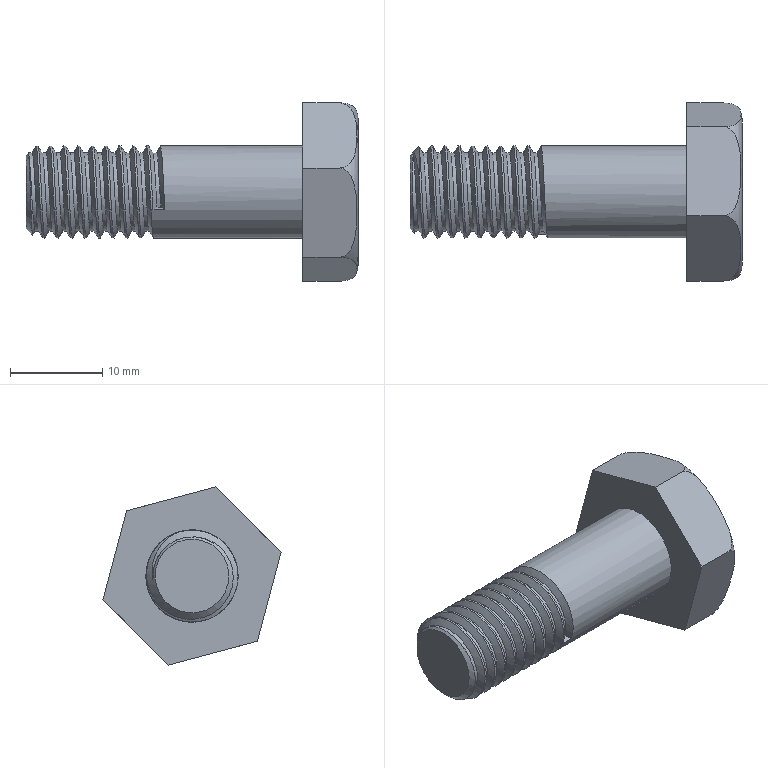Component | NX | CCJ-026_2 | 2 solids | 26 faces | volume 3718 mm3 | cylinder 11 | plane 11 | spline 2 | cone 1 | torus 1 | commonest cylinder face diameters 10 x10 8.5 x1